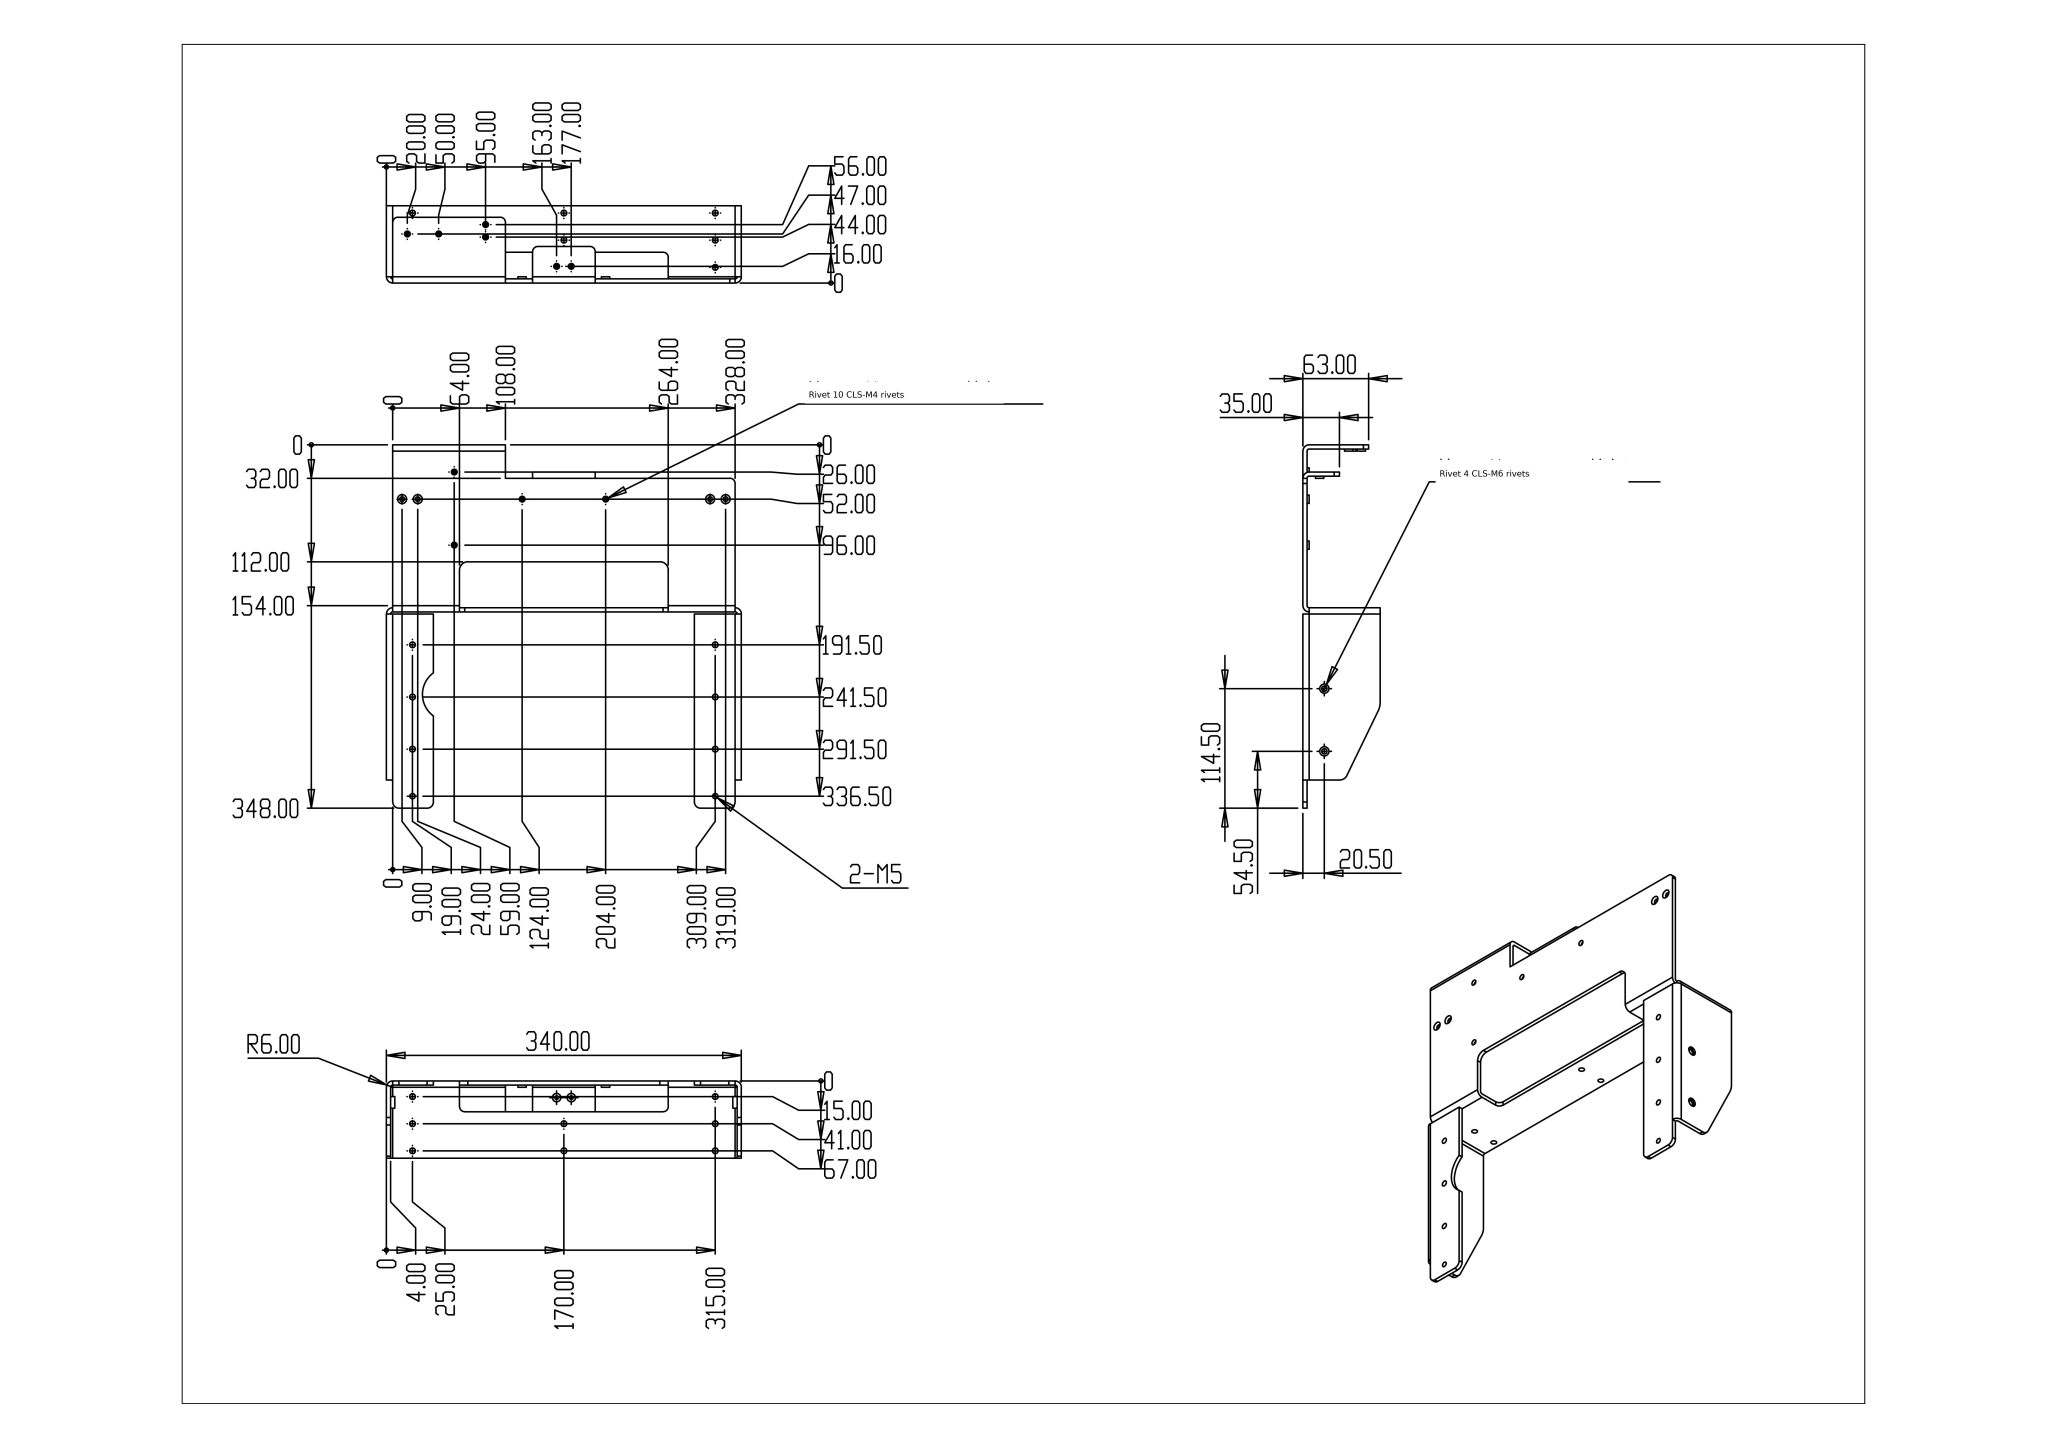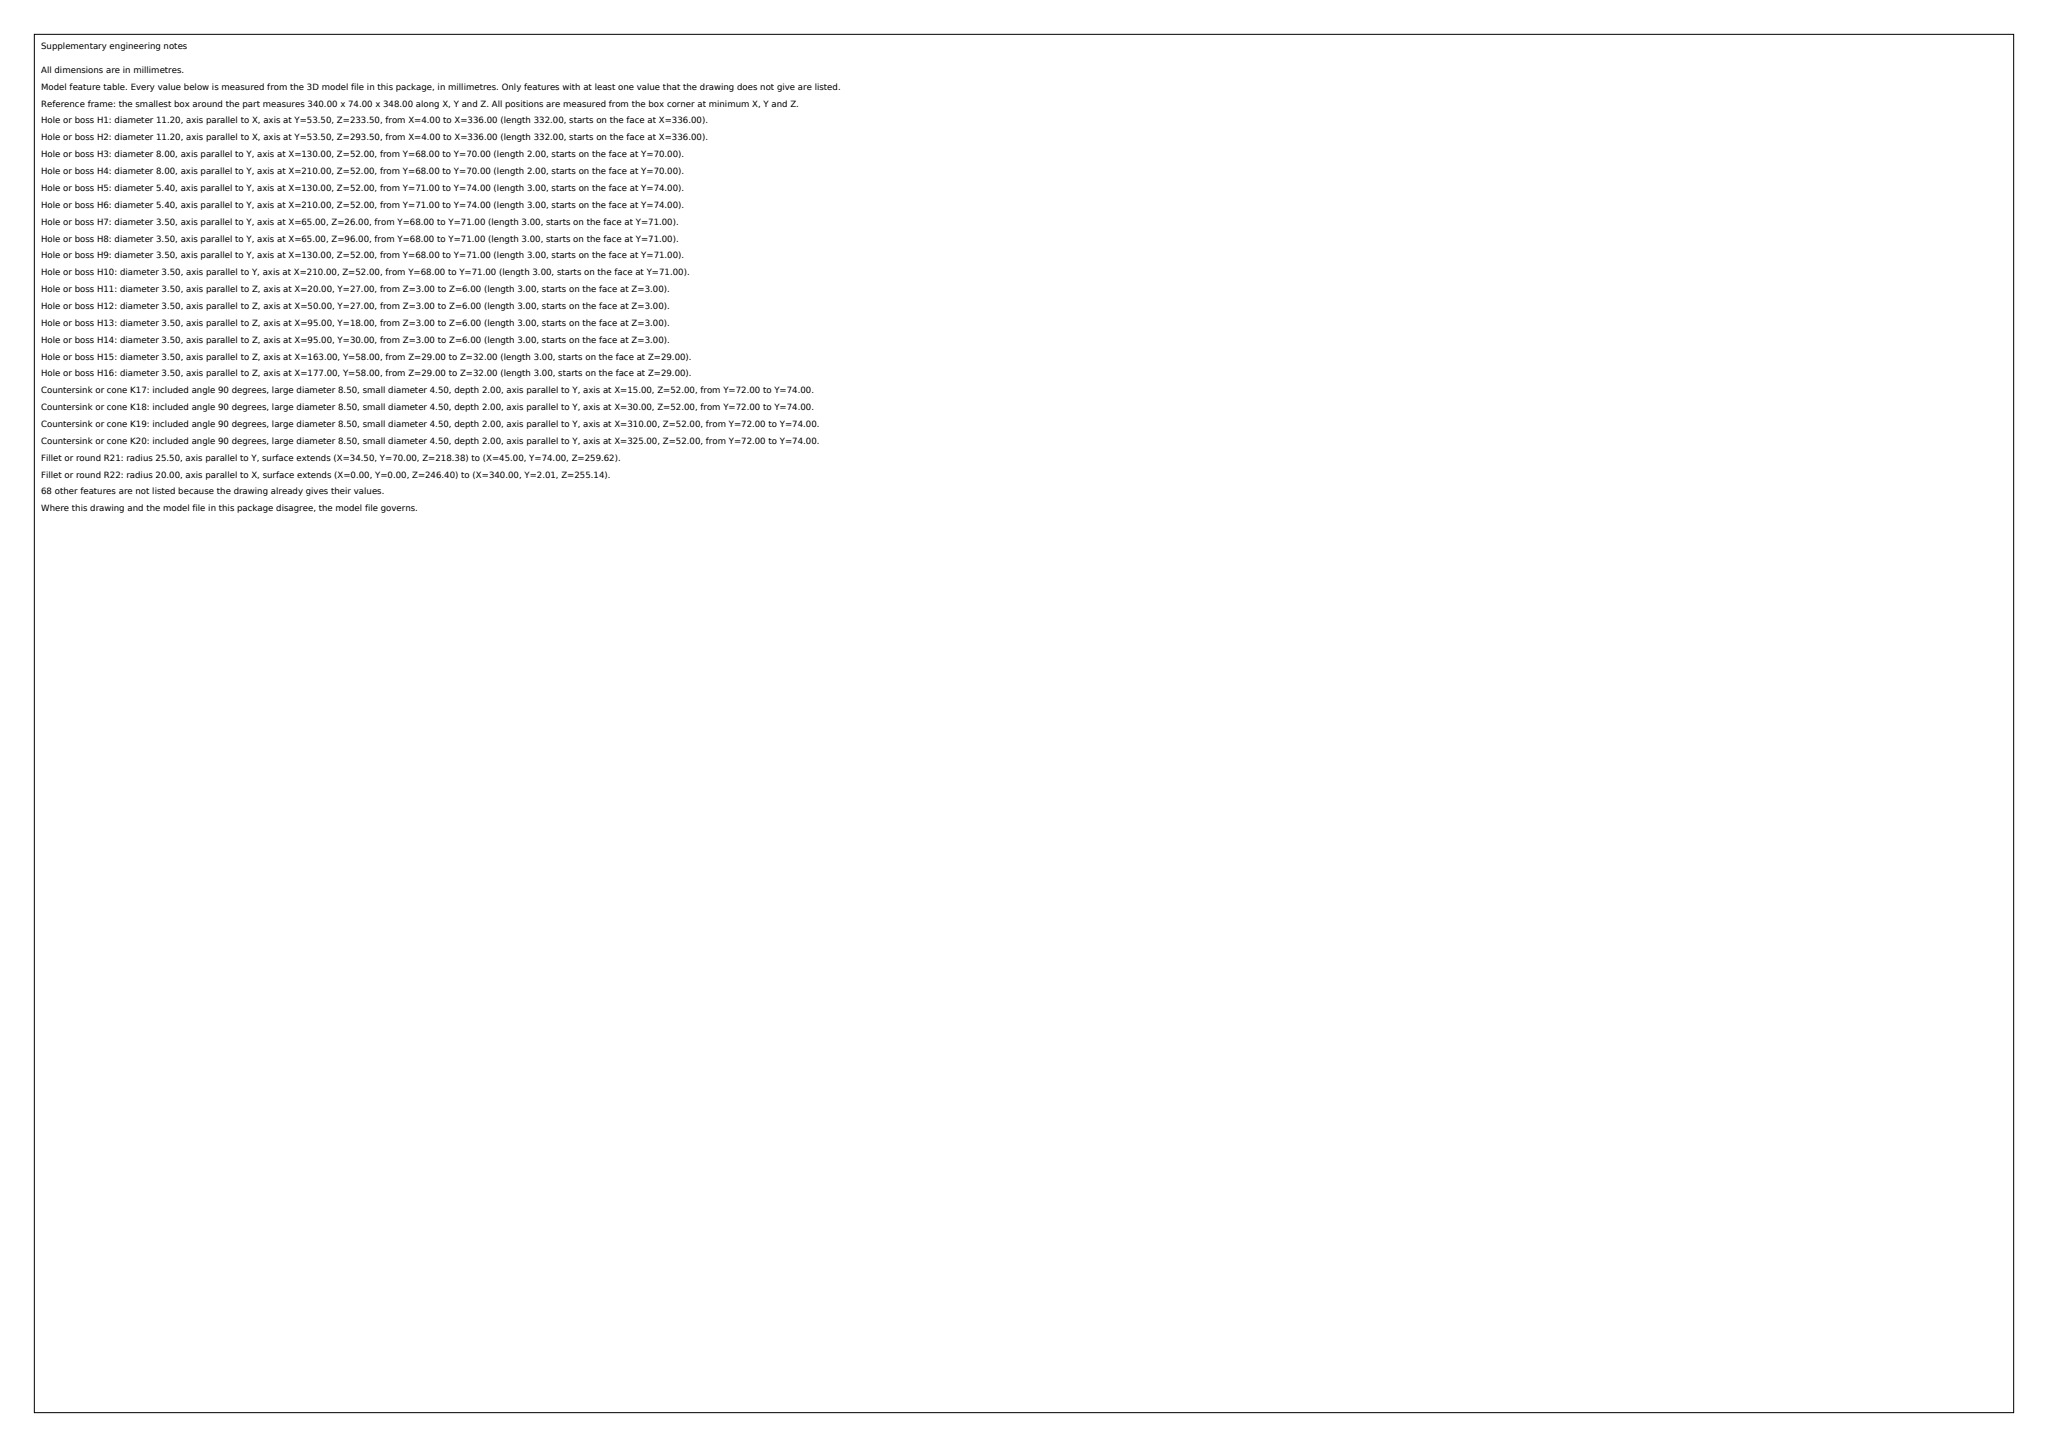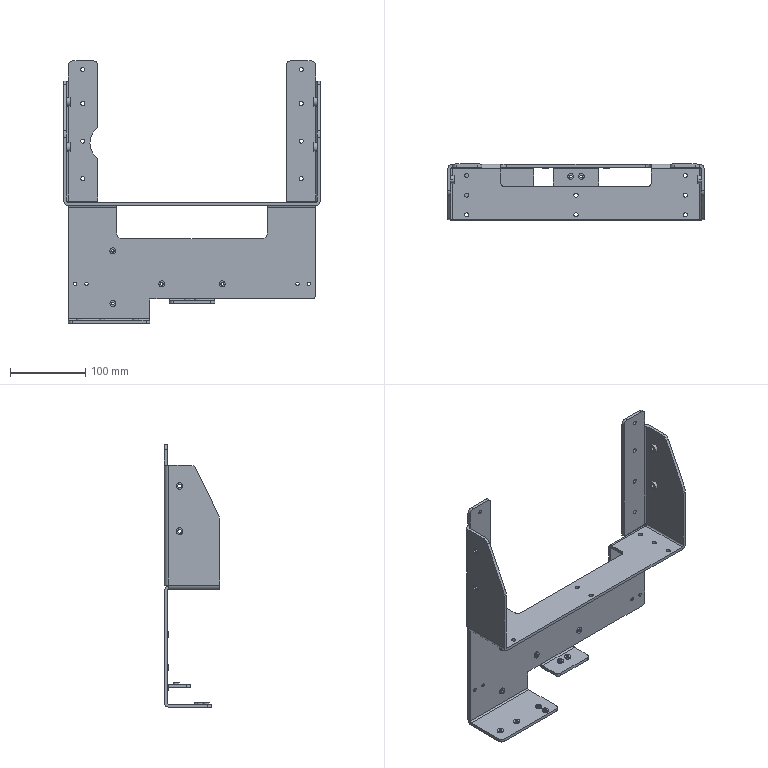Part | SolidWorks | mm | 1 solid | 239 faces | box 340 x 74 x 348 mm | volume 391028 mm3 | cylinder 158 | plane 73 | cone 8 | commonest cylinder face diameters 5.5 x28 3.5 x20 8 x20 5.41 x16 5 x12 12 x12 11.2 x8 4.5 x8